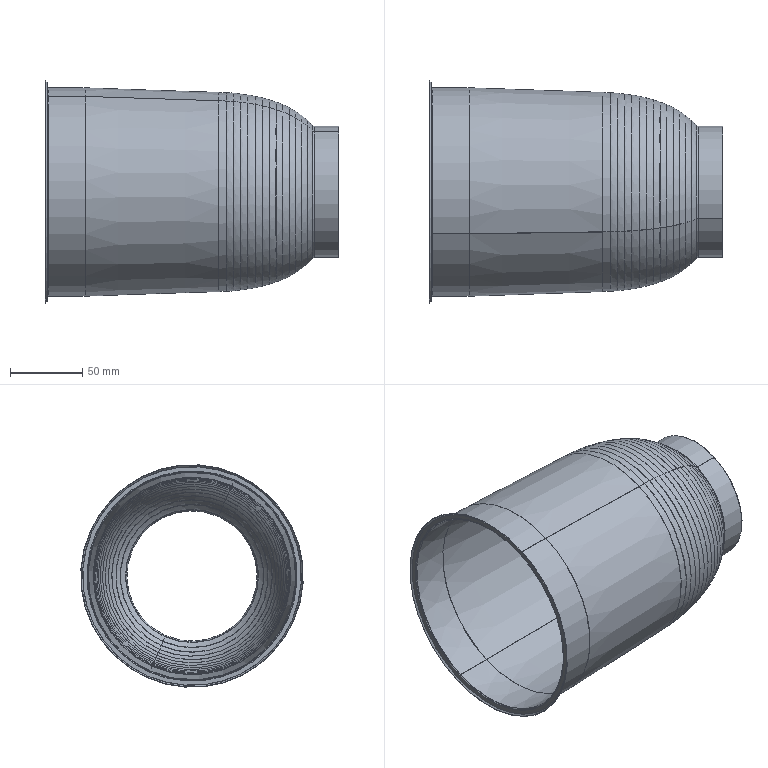Component | SolidWorks | EdgeTrimmingWorkpiece-2 | 1 solid | 85 faces | box 202.6 x 153.76 x 153.76 mm | volume 30622 mm3 | torus 60 | cone 16 | cylinder 6 | plane 3 | commonest cylinder face diameters 89.98 x2 90.68 x2 144.237 x2
build123d program:
from build123d import *


with BuildPart() as part:
    # Model → Revolve1 (revolve)
    with BuildSketch(Plane.XY, mode=Mode.PRIVATE) as revolve1_sk:
        with BuildLine():
            Line((15123.901, -1393.748), (15123.647, -1398.988))
            Line((15123.647, -1398.988), (15120.421, -1491.364))
            Line((15120.421, -1491.364), (15120.421, -1516.821))
            ThreePointArc((15120.421, -1516.821), (15120.275, -1517.175), (15119.921, -1517.321))
            Line((15119.921, -1517.321), (15116.819, -1517.321))
            Line((15116.819, -1517.321), (15115.659, -1518.481))
            Line((15115.659, -1518.481), (15115.942, -1518.764))
            Line((15115.942, -1518.764), (15117.041, -1517.665))
            Line((15117.041, -1517.665), (15119.921, -1517.665))
            ThreePointArc((15119.921, -1517.665), (15120.522, -1517.416), (15120.771, -1516.815))
            Line((15120.771, -1516.815), (15120.771, -1491.37))
            Line((15120.771, -1491.37), (15123.997, -1399.001))
            Line((15123.997, -1399.001), (15124.251, -1393.77))
            ThreePointArc((15124.251, -1393.77), (15124.424, -1391.273), (15124.634, -1388.78))
            ThreePointArc((15124.634, -1388.78), (15124.882, -1386.29), (15125.169, -1383.804))
            ThreePointArc((15125.169, -1383.804), (15125.497, -1381.323), (15125.869, -1378.849))
            ThreePointArc((15125.869, -1378.849), (15126.287, -1376.382), (15126.753, -1373.924))
            ThreePointArc((15126.753, -1373.924), (15127.269, -1371.476), (15127.839, -1369.04))
            ThreePointArc((15127.839, -1369.04), (15128.465, -1366.618), (15129.151, -1364.213))
            ThreePointArc((15129.151, -1364.213), (15129.898, -1361.827), (15130.711, -1359.462))
            ThreePointArc((15130.711, -1359.462), (15131.593, -1357.123), (15132.547, -1354.813))
            ThreePointArc((15132.547, -1354.813), (15133.577, -1352.538), (15134.686, -1350.301))
            ThreePointArc((15134.686, -1350.301), (15135.876, -1348.11), (15137.152, -1345.967))
            ThreePointArc((15137.152, -1345.967), (15138.514, -1343.885), (15139.966, -1341.865))
            ThreePointArc((15139.966, -1341.865), (15141.53, -1339.889), (15143.19, -1337.993))
            ThreePointArc((15143.19, -1337.993), (15144.934, -1336.194), (15146.77, -1334.489))
            ThreePointArc((15146.77, -1334.489), (15147.346, -1333.71), (15147.55, -1332.763))
            Line((15147.55, -1332.763), (15147.55, -1316.165))
            Line((15147.55, -1316.165), (15147.2, -1316.165))
            Line((15147.2, -1316.165), (15147.2, -1332.763))
            ThreePointArc((15147.2, -1332.763), (15147.027, -1333.566), (15146.539, -1334.226))
            ThreePointArc((15146.539, -1334.226), (15144.689, -1335.944), (15142.933, -1337.756))
            ThreePointArc((15142.933, -1337.756), (15141.261, -1339.665), (15139.686, -1341.654))
            ThreePointArc((15139.686, -1341.654), (15138.225, -1343.687), (15136.855, -1345.782))
            ThreePointArc((15136.855, -1345.782), (15135.572, -1347.937), (15134.375, -1350.14))
            ThreePointArc((15134.375, -1350.14), (15133.261, -1352.389), (15132.226, -1354.675))
            ThreePointArc((15132.226, -1354.675), (15131.267, -1356.995), (15130.382, -1359.344))
            ThreePointArc((15130.382, -1359.344), (15129.566, -1361.717), (15128.815, -1364.113))
            ThreePointArc((15128.815, -1364.113), (15128.128, -1366.527), (15127.499, -1368.957))
            ThreePointArc((15127.499, -1368.957), (15126.928, -1371.4), (15126.41, -1373.855))
            ThreePointArc((15126.41, -1373.855), (15125.942, -1376.32), (15125.524, -1378.794))
            ThreePointArc((15125.524, -1378.794), (15125.151, -1381.274), (15124.821, -1383.761))
            ThreePointArc((15124.821, -1383.761), (15124.534, -1386.252), (15124.286, -1388.748))
            ThreePointArc((15124.286, -1388.748), (15124.076, -1391.247), (15123.901, -1393.748))
        make_face()
    revolve(revolve1_sk.sketch.rotate(Axis((15192.54, -1249.447, 0), (0, -1, 0)), 270), axis=Axis((15192.54, -1249.447, 0), (0, -1, 0)))


solid = part.part

# Placed as in the assembly
solid = solid.moved(Location((1497.626, 16492.246, 687.116), (0, 0, -90)))